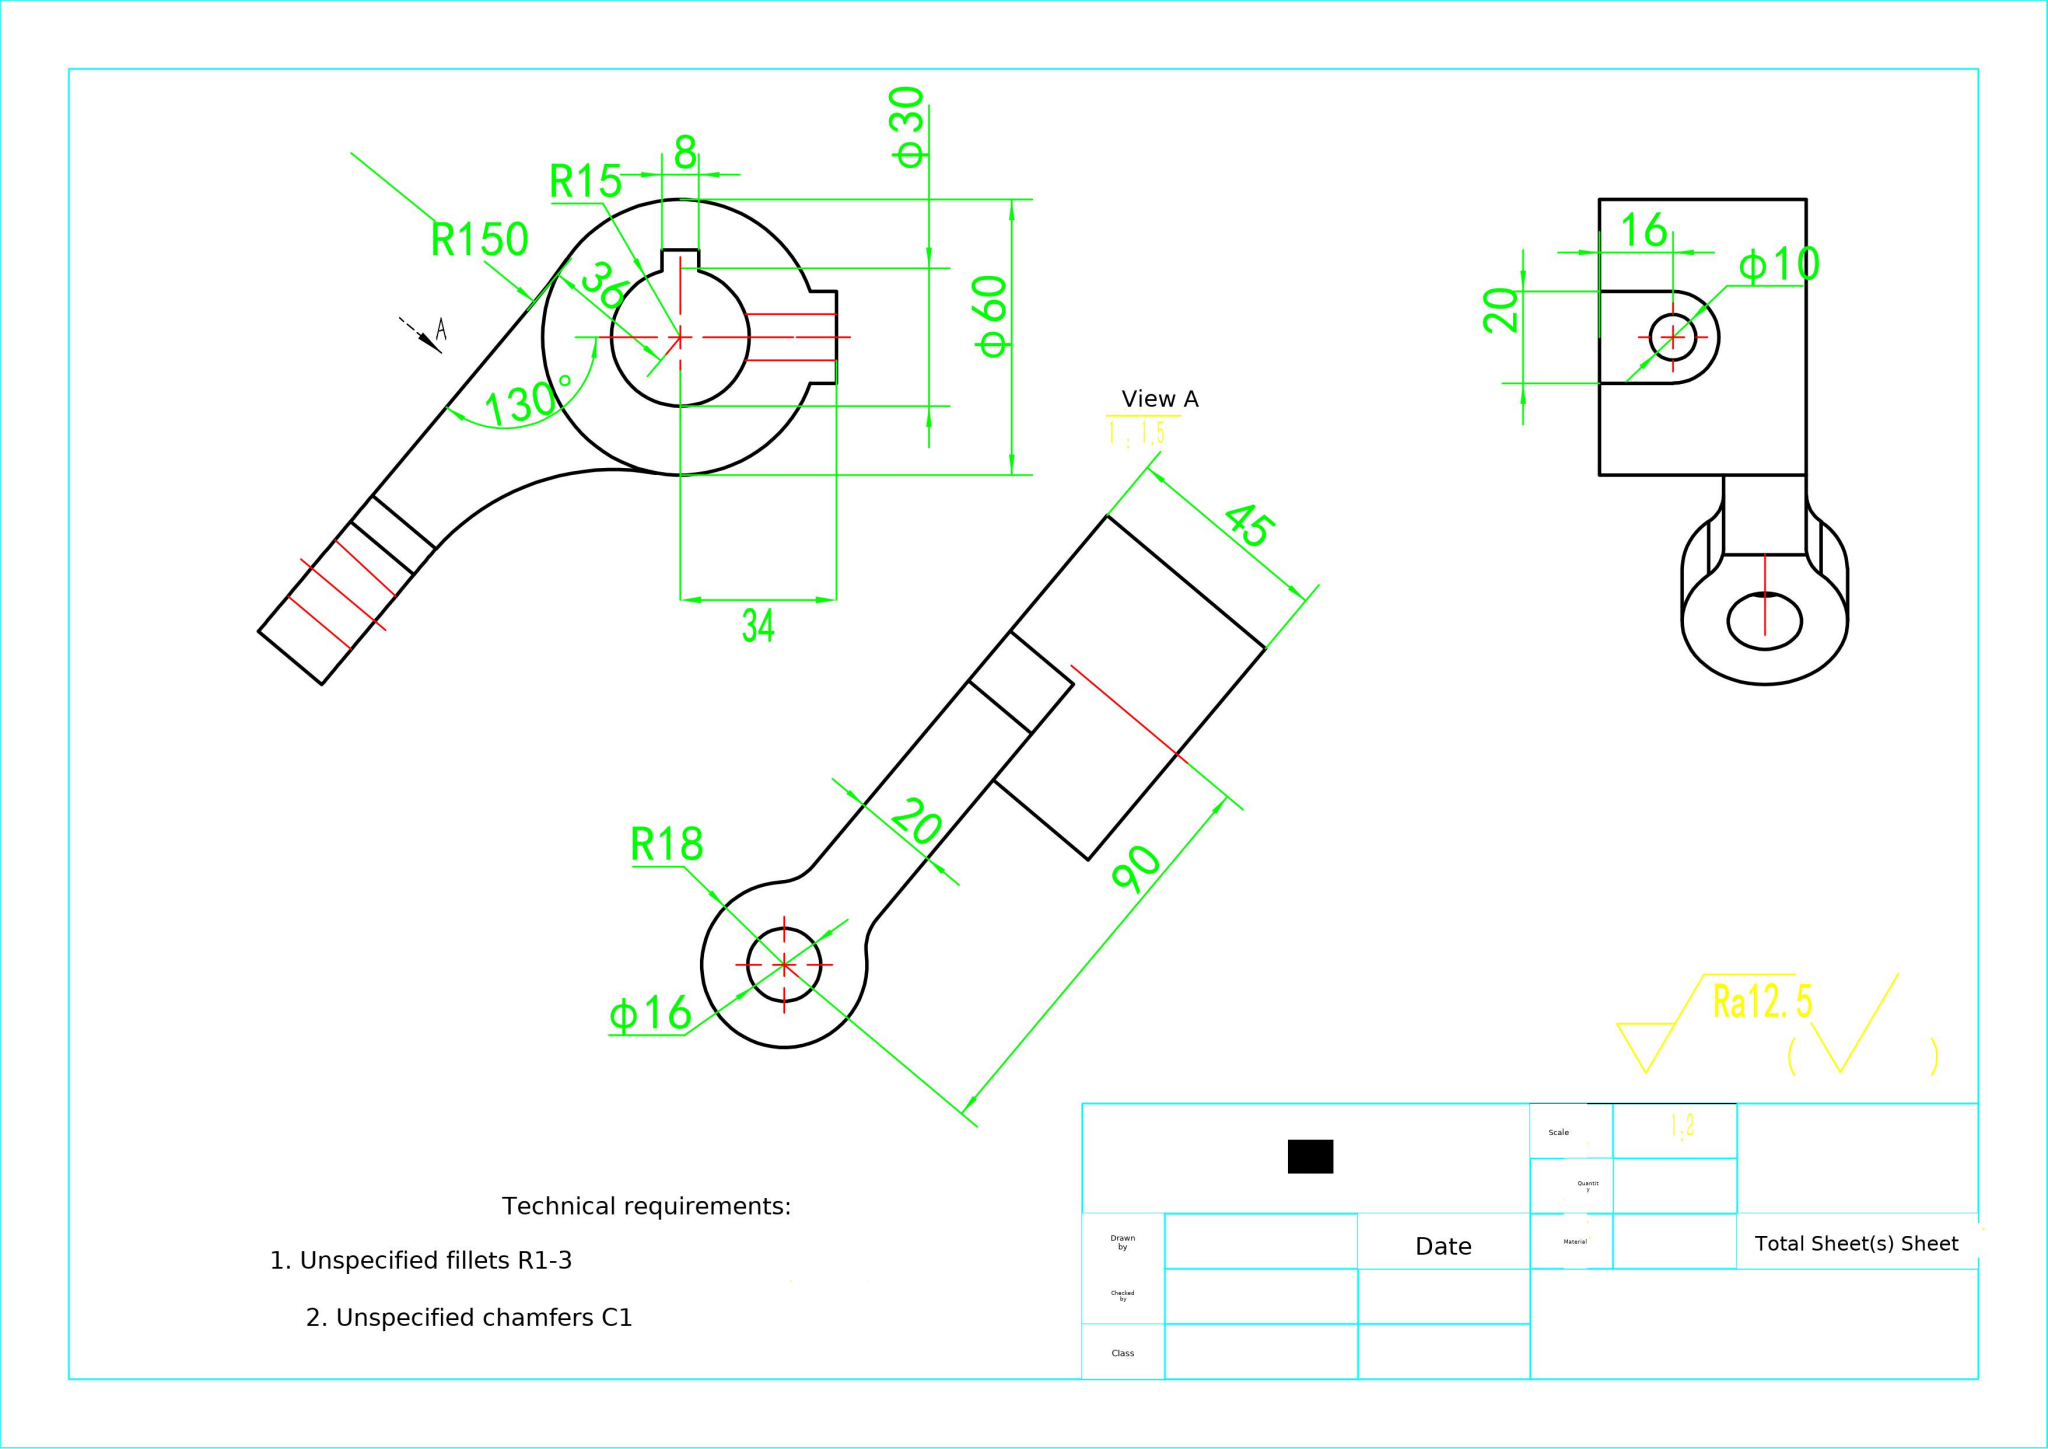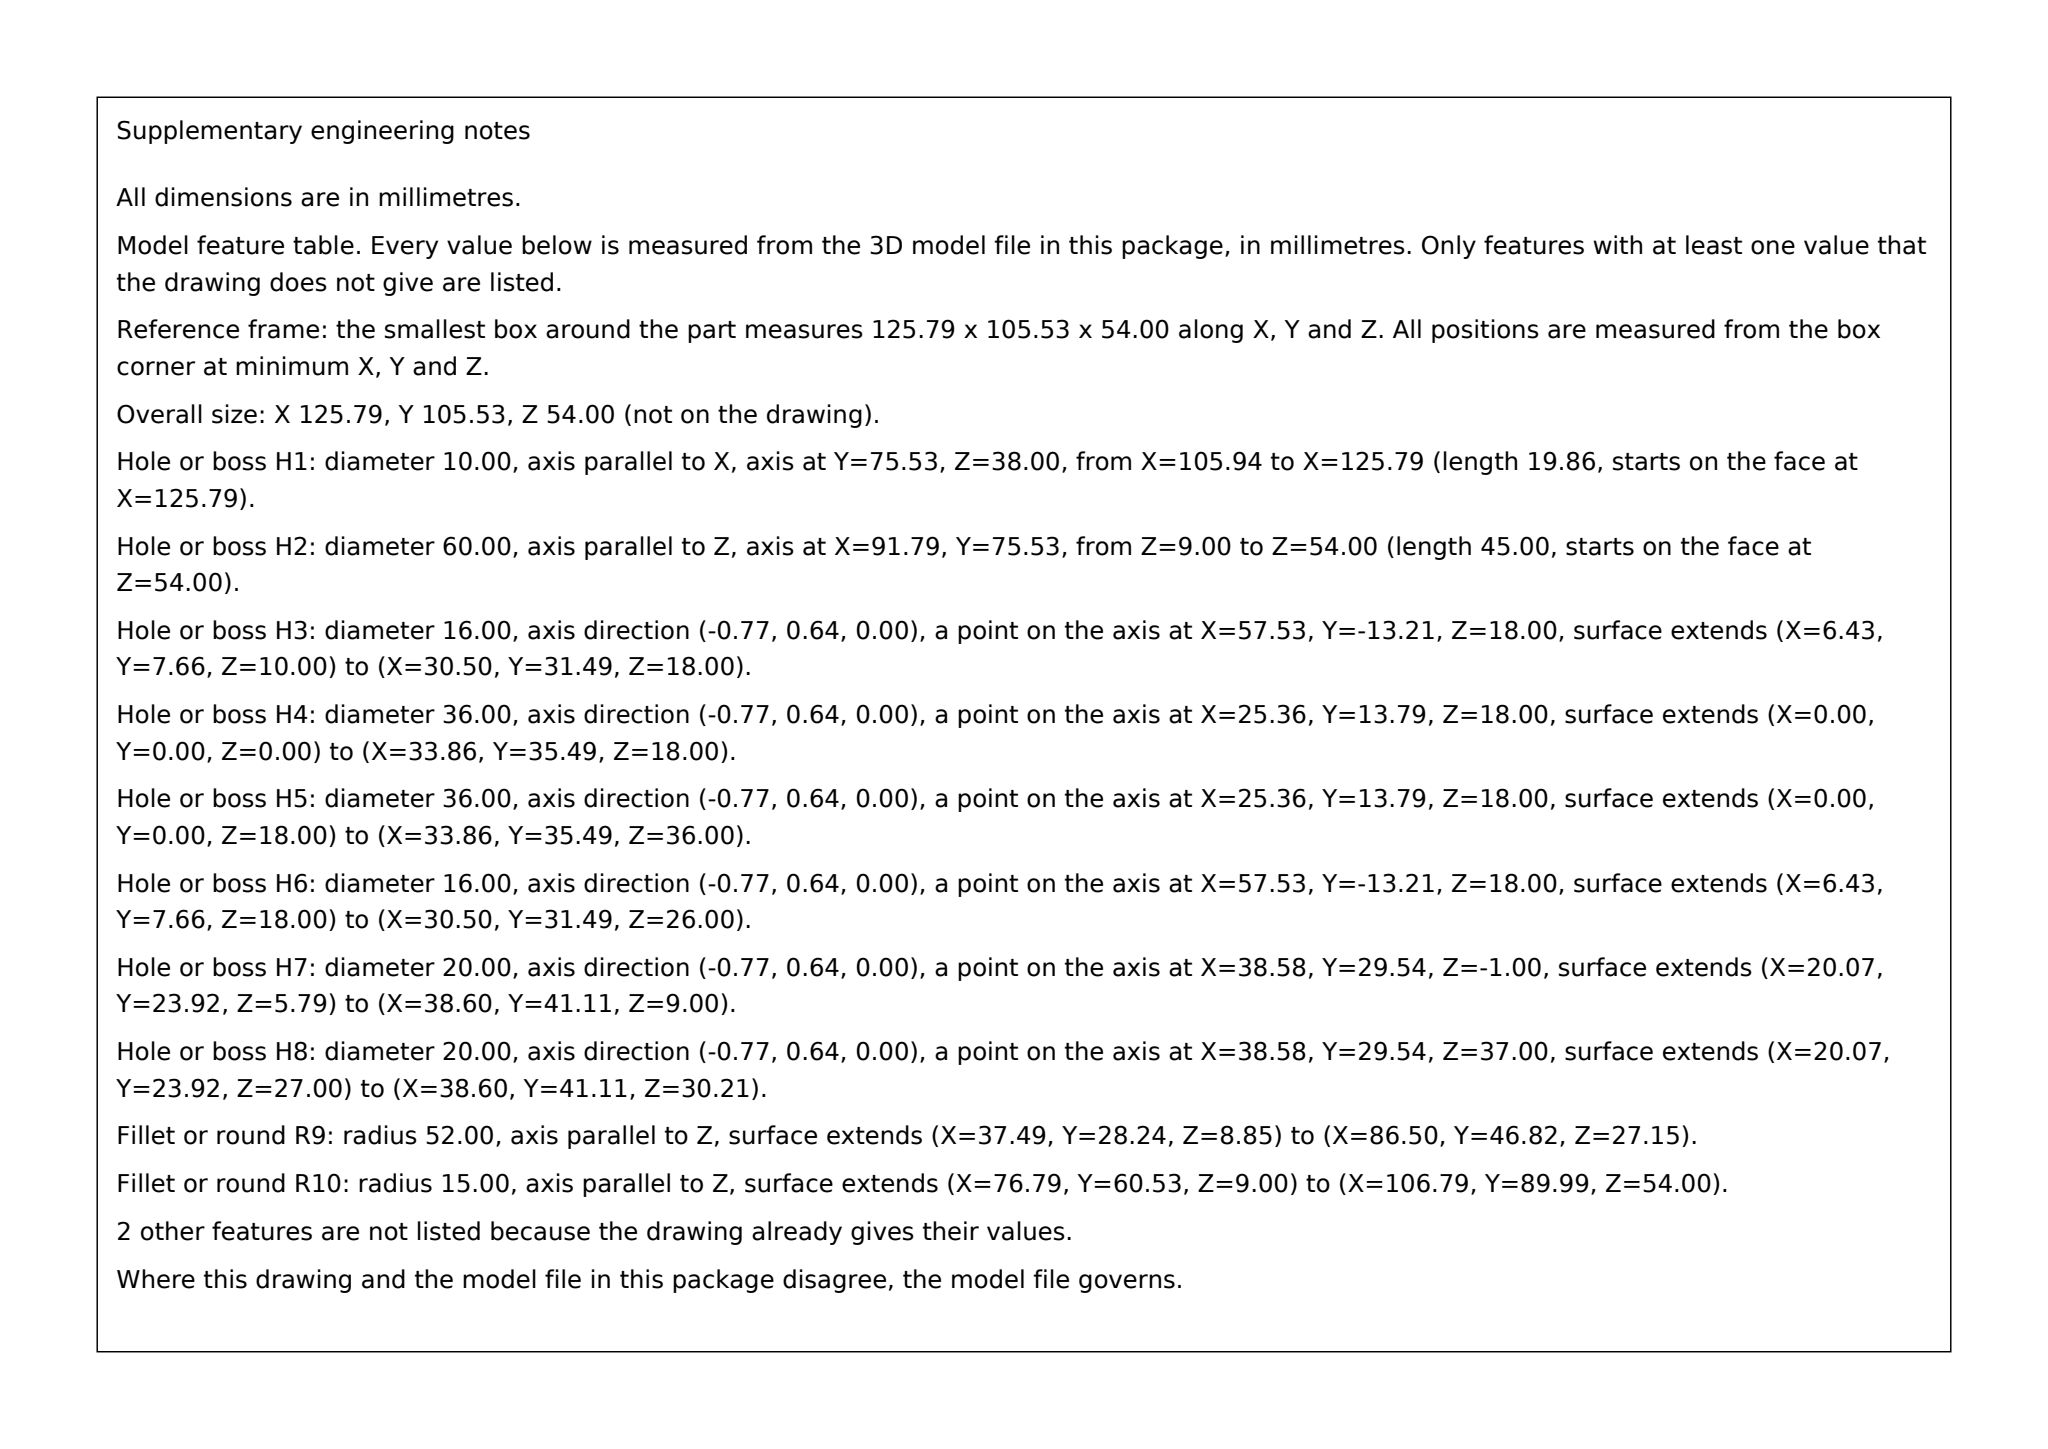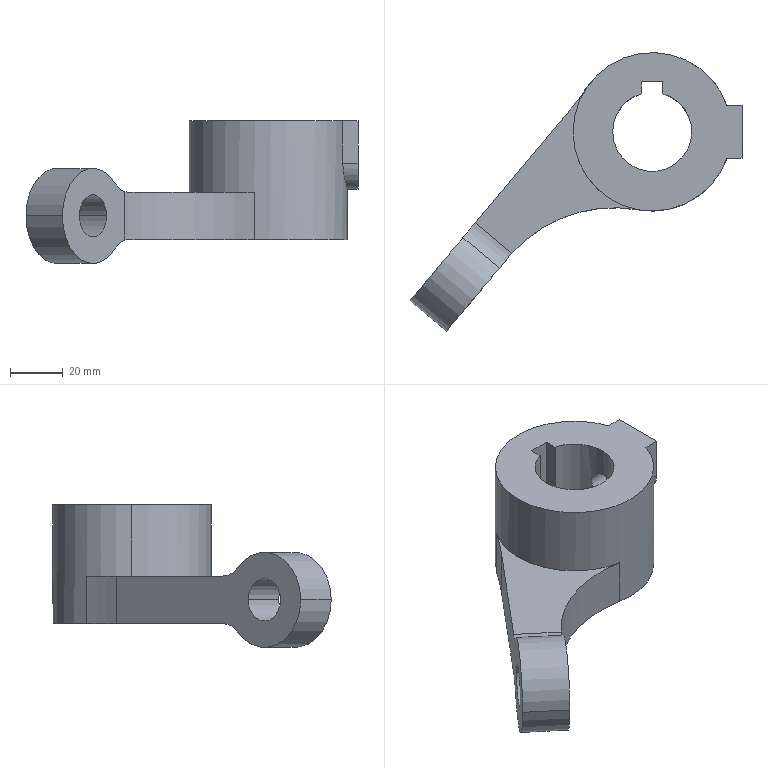Part | SolidWorks | mm | 1 solid | 28 faces | box 125.79 x 105.53 x 54 mm | volume 131027 mm3 | cylinder 17 | plane 11 | commonest cylinder face diameters 20 x4 30 x3 10 x2 16 x2 36 x2 60 x2 300 x1 104 x1